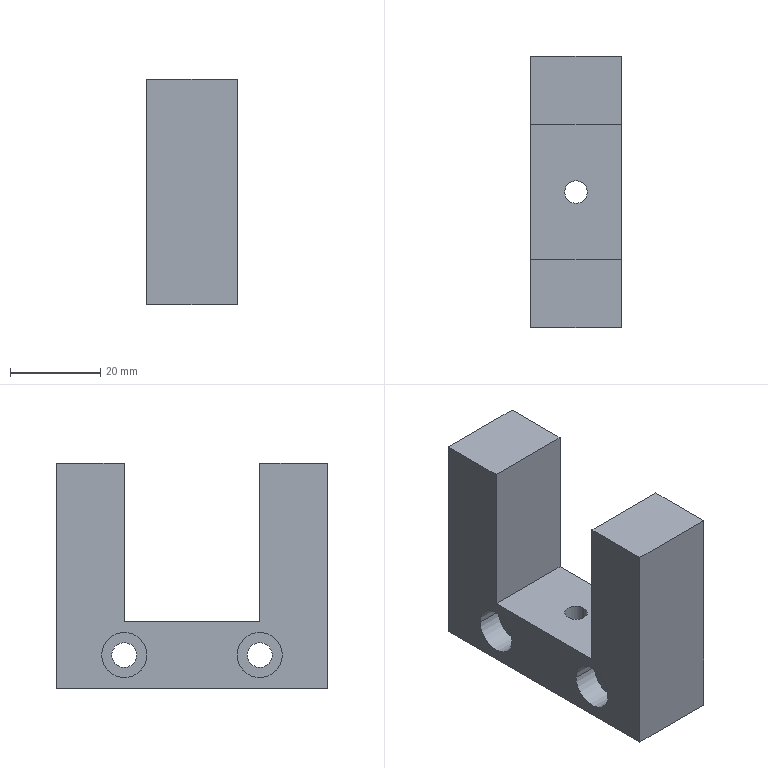Component | SolidWorks | LongSideClampingAssemblyBGeneralAssembly-1_LimitB-0510-1 | 1 solid | 22 faces | box 20 x 60 x 50 mm | volume 37131 mm3 | plane 12 | cylinder 10 | commonest cylinder face diameters 10 x4 5.5 x4 5 x2 | material Q235-A
build123d program:
from build123d import *

# Parameters (mm, degrees)
BOSS_EXTRUDE1_DEPTH                                = 20
HOLE_SIZE_ACCORDING_TO_TYPE_OF_HEX_SOC_D           = 5.5
HOLE_SIZE_ACCORDING_TO_TYPE_OF_HEX_SOC_CBORE_D     = 10
HOLE_SIZE_ACCORDING_TO_TYPE_OF_HEX_SOC_CBORE_DEPTH = 5.7
M6_TAPPED_HOLE1_D                                  = 5


with BuildPart() as part:
    # Sketch1 → Boss-Extrude1 (new body)
    with BuildSketch(Plane.XY):
        Polygon((-30, -25), (-15, -25), (-15, 10), (15, 10), (15, -25), (30, -25), (30, 25), (-30, 25), align=None)
    extrude(amount=BOSS_EXTRUDE1_DEPTH)

    # Hole Size _According to_ Type of Hex Soc (through all)
    with Locations(Plane.XY.offset(20)):
        with Locations((-15, 17.5), (15, 17.5)):
            CounterBoreHole(HOLE_SIZE_ACCORDING_TO_TYPE_OF_HEX_SOC_D / 2, HOLE_SIZE_ACCORDING_TO_TYPE_OF_HEX_SOC_CBORE_D / 2, HOLE_SIZE_ACCORDING_TO_TYPE_OF_HEX_SOC_CBORE_DEPTH)

    # M6 Tapped Hole1 (through all)
    with Locations(Plane(origin=(0, 25, 0), x_dir=(1, 0, 0), z_dir=(0, 1, 0))):
        with Locations((0, -10)):
            Hole(M6_TAPPED_HOLE1_D / 2)


solid = part.part

# Placed as in the assembly
solid = solid.moved(Location((-3220.658, 0.3914, 3511), (-90, -90, 0)))
STEP:
#1=CARTESIAN_POINT('',(-127.093,0.01541,137.835));
#2=VERTEX_POINT('',#1);
#3=CARTESIAN_POINT('',(-127.29,0.01541,137.835));
#4=VERTEX_POINT('',#3);
#5=CARTESIAN_POINT('',(-127.191,0.01541,137.835));
#6=DIRECTION('',(-0.,-0.,-1.));
#7=DIRECTION('',(0.,-1.,0.));
#8=AXIS2_PLACEMENT_3D('',#5,#6,#7);
#9=CIRCLE('',#8,0.09843);
#10=EDGE_CURVE('',#2,#4,#9,.T.);
#11=ORIENTED_EDGE('',*,*,#10,.F.);
#12=CARTESIAN_POINT('',(-127.093,0.01541,137.244));
#13=VERTEX_POINT('',#12);
#14=CARTESIAN_POINT('',(-127.093,0.01541,137.244));
#15=DIRECTION('',(-0.,-0.,-1.));
#16=VECTOR('',#15,39.37);
#17=LINE('',#14,#16);
#18=EDGE_CURVE('',#2,#13,#17,.T.);
#19=ORIENTED_EDGE('',*,*,#18,.T.);
#20=CARTESIAN_POINT('',(-127.29,0.01541,137.244));
#21=VERTEX_POINT('',#20);
#22=CARTESIAN_POINT('',(-127.191,0.01541,137.244));
#23=DIRECTION('',(-0.,-0.,-1.));
#24=DIRECTION('',(-1.,0.,0.));
#25=AXIS2_PLACEMENT_3D('',#22,#23,#24);
#26=CIRCLE('',#25,0.09843);
#27=EDGE_CURVE('',#13,#21,#26,.T.);
#28=ORIENTED_EDGE('',*,*,#27,.T.);
#29=CARTESIAN_POINT('',(-127.29,0.01541,137.244));
#30=DIRECTION('',(-0.,-0.,-1.));
#31=VECTOR('',#30,39.37);
#32=LINE('',#29,#31);
#33=EDGE_CURVE('',#4,#21,#32,.T.);
#34=ORIENTED_EDGE('',*,*,#33,.F.);
#35=EDGE_LOOP('',(#11,#19,#28,#34));
#36=FACE_OUTER_BOUND('',#35,.T.);
#37=CARTESIAN_POINT('',(-127.191,0.01541,137.244));
#38=DIRECTION('',(-0.,-0.,-1.));
#39=DIRECTION('',(-1.,0.,0.));
#40=AXIS2_PLACEMENT_3D('',#37,#38,#39);
#41=CYLINDRICAL_SURFACE('',#40,0.09843);
#42=ADVANCED_FACE('',(#36),#41,.F.);
#43=CARTESIAN_POINT('',(-127.361,-0.772,137.539));
#44=VERTEX_POINT('',#43);
#45=CARTESIAN_POINT('',(-127.361,-0.3783,137.539));
#46=VERTEX_POINT('',#45);
#47=CARTESIAN_POINT('',(-127.361,-0.5751,137.539));
#48=DIRECTION('',(-1.,0.,0.));
#49=DIRECTION('',(0.,1.,0.));
#50=AXIS2_PLACEMENT_3D('',#47,#48,#49);
#51=CIRCLE('',#50,0.1969);
#52=EDGE_CURVE('',#44,#46,#51,.T.);
#53=ORIENTED_EDGE('',*,*,#52,.F.);
#54=CARTESIAN_POINT('',(-127.585,-0.772,137.539));
#55=VERTEX_POINT('',#54);
#56=CARTESIAN_POINT('',(-127.585,-0.772,137.539));
#57=DIRECTION('',(-1.,0.,0.));
#58=VECTOR('',#57,39.37);
#59=LINE('',#56,#58);
#60=EDGE_CURVE('',#44,#55,#59,.T.);
#61=ORIENTED_EDGE('',*,*,#60,.T.);
#62=CARTESIAN_POINT('',(-127.585,-0.3783,137.539));
#63=VERTEX_POINT('',#62);
#64=CARTESIAN_POINT('',(-127.585,-0.5751,137.539));
#65=DIRECTION('',(-1.,0.,0.));
#66=DIRECTION('',(0.,1.,0.));
#67=AXIS2_PLACEMENT_3D('',#64,#65,#66);
#68=CIRCLE('',#67,0.1969);
#69=EDGE_CURVE('',#55,#63,#68,.T.);
#70=ORIENTED_EDGE('',*,*,#69,.T.);
#71=CARTESIAN_POINT('',(-127.585,-0.3783,137.539));
#72=DIRECTION('',(-1.,0.,0.));
#73=VECTOR('',#72,39.37);
#74=LINE('',#71,#73);
#75=EDGE_CURVE('',#46,#63,#74,.T.);
#76=ORIENTED_EDGE('',*,*,#75,.F.);
#77=EDGE_LOOP('',(#53,#61,#70,#76));
#78=FACE_OUTER_BOUND('',#77,.T.);
#79=CARTESIAN_POINT('',(-127.585,-0.5751,137.539));
#80=DIRECTION('',(-1.,0.,0.));
#81=DIRECTION('',(0.,1.,0.));
#82=AXIS2_PLACEMENT_3D('',#79,#80,#81);
#83=CYLINDRICAL_SURFACE('',#82,0.1969);
#84=ADVANCED_FACE('',(#78),#83,.F.);
#85=CARTESIAN_POINT('',(-126.798,-0.6834,137.539));
#86=VERTEX_POINT('',#85);
#87=CARTESIAN_POINT('',(-126.798,-0.4669,137.539));
#88=VERTEX_POINT('',#87);
#89=CARTESIAN_POINT('',(-126.798,-0.5751,137.539));
#90=DIRECTION('',(-1.,0.,0.));
#91=DIRECTION('',(0.,1.,0.));
#92=AXIS2_PLACEMENT_3D('',#89,#90,#91);
#93=CIRCLE('',#92,0.1083);
#94=EDGE_CURVE('',#86,#88,#93,.T.);
#95=ORIENTED_EDGE('',*,*,#94,.F.);
#96=CARTESIAN_POINT('',(-127.361,-0.6834,137.539));
#97=VERTEX_POINT('',#96);
#98=CARTESIAN_POINT('',(-127.585,-0.6834,137.539));
#99=DIRECTION('',(-1.,0.,0.));
#100=VECTOR('',#99,39.37);
#101=LINE('',#98,#100);
#102=EDGE_CURVE('',#86,#97,#101,.T.);
#103=ORIENTED_EDGE('',*,*,#102,.T.);
#104=CARTESIAN_POINT('',(-127.361,-0.4669,137.539));
#105=VERTEX_POINT('',#104);
#106=CARTESIAN_POINT('',(-127.361,-0.5751,137.539));
#107=DIRECTION('',(-1.,0.,0.));
#108=DIRECTION('',(0.,1.,0.));
#109=AXIS2_PLACEMENT_3D('',#106,#107,#108);
#110=CIRCLE('',#109,0.1083);
#111=EDGE_CURVE('',#97,#105,#110,.T.);
#112=ORIENTED_EDGE('',*,*,#111,.T.);
#113=CARTESIAN_POINT('',(-127.585,-0.4669,137.539));
#114=DIRECTION('',(-1.,0.,0.));
#115=VECTOR('',#114,39.37);
#116=LINE('',#113,#115);
#117=EDGE_CURVE('',#88,#105,#116,.T.);
#118=ORIENTED_EDGE('',*,*,#117,.F.);
#119=EDGE_LOOP('',(#95,#103,#112,#118));
#120=FACE_OUTER_BOUND('',#119,.T.);
#121=CARTESIAN_POINT('',(-127.585,-0.5751,137.539));
#122=DIRECTION('',(-1.,0.,0.));
#123=DIRECTION('',(0.,1.,0.));
#124=AXIS2_PLACEMENT_3D('',#121,#122,#123);
#125=CYLINDRICAL_SURFACE('',#124,0.1083);
#126=ADVANCED_FACE('',(#120),#125,.F.);
#127=CARTESIAN_POINT('',(-127.361,0.4091,137.539));
#128=VERTEX_POINT('',#127);
#129=CARTESIAN_POINT('',(-127.361,0.8028,137.539));
#130=VERTEX_POINT('',#129);
#131=CARTESIAN_POINT('',(-127.361,0.606,137.539));
#132=DIRECTION('',(-1.,0.,0.));
#133=DIRECTION('',(0.,1.,0.));
#134=AXIS2_PLACEMENT_3D('',#131,#132,#133);
#135=CIRCLE('',#134,0.1969);
#136=EDGE_CURVE('',#128,#130,#135,.T.);
#137=ORIENTED_EDGE('',*,*,#136,.F.);
#138=CARTESIAN_POINT('',(-127.585,0.4091,137.539));
#139=VERTEX_POINT('',#138);
#140=CARTESIAN_POINT('',(-127.585,0.4091,137.539));
#141=DIRECTION('',(-1.,0.,0.));
#142=VECTOR('',#141,39.37);
#143=LINE('',#140,#142);
#144=EDGE_CURVE('',#128,#139,#143,.T.);
#145=ORIENTED_EDGE('',*,*,#144,.T.);
#146=CARTESIAN_POINT('',(-127.585,0.8028,137.539));
#147=VERTEX_POINT('',#146);
#148=CARTESIAN_POINT('',(-127.585,0.606,137.539));
#149=DIRECTION('',(-1.,0.,0.));
#150=DIRECTION('',(0.,1.,0.));
#151=AXIS2_PLACEMENT_3D('',#148,#149,#150);
#152=CIRCLE('',#151,0.1969);
#153=EDGE_CURVE('',#139,#147,#152,.T.);
#154=ORIENTED_EDGE('',*,*,#153,.T.);
#155=CARTESIAN_POINT('',(-127.585,0.8028,137.539));
#156=DIRECTION('',(-1.,0.,0.));
#157=VECTOR('',#156,39.37);
#158=LINE('',#155,#157);
#159=EDGE_CURVE('',#130,#147,#158,.T.);
#160=ORIENTED_EDGE('',*,*,#159,.F.);
#161=EDGE_LOOP('',(#137,#145,#154,#160));
#162=FACE_OUTER_BOUND('',#161,.T.);
#163=CARTESIAN_POINT('',(-127.585,0.606,137.539));
#164=DIRECTION('',(-1.,0.,0.));
#165=DIRECTION('',(0.,1.,0.));
#166=AXIS2_PLACEMENT_3D('',#163,#164,#165);
#167=CYLINDRICAL_SURFACE('',#166,0.1969);
#168=ADVANCED_FACE('',(#162),#167,.F.);
#169=CARTESIAN_POINT('',(-126.798,0.4977,137.539));
#170=VERTEX_POINT('',#169);
#171=CARTESIAN_POINT('',(-126.798,0.7142,137.539));
#172=VERTEX_POINT('',#171);
#173=CARTESIAN_POINT('',(-126.798,0.606,137.539));
#174=DIRECTION('',(-1.,0.,0.));
#175=DIRECTION('',(0.,1.,0.));
#176=AXIS2_PLACEMENT_3D('',#173,#174,#175);
#177=CIRCLE('',#176,0.1083);
#178=EDGE_CURVE('',#170,#172,#177,.T.);
#179=ORIENTED_EDGE('',*,*,#178,.F.);
#180=CARTESIAN_POINT('',(-127.361,0.4977,137.539));
#181=VERTEX_POINT('',#180);
#182=CARTESIAN_POINT('',(-127.585,0.4977,137.539));
#183=DIRECTION('',(-1.,0.,0.));
#184=VECTOR('',#183,39.37);
#185=LINE('',#182,#184);
#186=EDGE_CURVE('',#170,#181,#185,.T.);
#187=ORIENTED_EDGE('',*,*,#186,.T.);
#188=CARTESIAN_POINT('',(-127.361,0.7142,137.539));
#189=VERTEX_POINT('',#188);
#190=CARTESIAN_POINT('',(-127.361,0.606,137.539));
#191=DIRECTION('',(-1.,0.,0.));
#192=DIRECTION('',(0.,1.,0.));
#193=AXIS2_PLACEMENT_3D('',#190,#191,#192);
#194=CIRCLE('',#193,0.1083);
#195=EDGE_CURVE('',#181,#189,#194,.T.);
#196=ORIENTED_EDGE('',*,*,#195,.T.);
#197=CARTESIAN_POINT('',(-127.585,0.7142,137.539));
#198=DIRECTION('',(-1.,0.,0.));
#199=VECTOR('',#198,39.37);
#200=LINE('',#197,#199);
#201=EDGE_CURVE('',#172,#189,#200,.T.);
#202=ORIENTED_EDGE('',*,*,#201,.F.);
#203=EDGE_LOOP('',(#179,#187,#196,#202));
#204=FACE_OUTER_BOUND('',#203,.T.);
#205=CARTESIAN_POINT('',(-127.585,0.606,137.539));
#206=DIRECTION('',(-1.,0.,0.));
#207=DIRECTION('',(0.,1.,0.));
#208=AXIS2_PLACEMENT_3D('',#205,#206,#207);
#209=CYLINDRICAL_SURFACE('',#208,0.1083);
#210=ADVANCED_FACE('',(#204),#209,.F.);
#211=CARTESIAN_POINT('',(-126.798,1.197,139.213));
#212=VERTEX_POINT('',#211);
#213=CARTESIAN_POINT('',(-126.798,1.197,137.244));
#214=VERTEX_POINT('',#213);
#215=CARTESIAN_POINT('',(-126.798,1.197,139.213));
#216=DIRECTION('',(-0.,0.,-1.));
#217=VECTOR('',#216,39.37);
#218=LINE('',#215,#217);
#219=EDGE_CURVE('',#212,#214,#218,.T.);
#220=ORIENTED_EDGE('',*,*,#219,.T.);
#221=CARTESIAN_POINT('',(-127.585,1.197,137.244));
#222=VERTEX_POINT('',#221);
#223=CARTESIAN_POINT('',(-127.585,1.197,137.244));
#224=DIRECTION('',(1.,-0.,-0.));
#225=VECTOR('',#224,39.37);
#226=LINE('',#223,#225);
#227=EDGE_CURVE('',#222,#214,#226,.T.);
#228=ORIENTED_EDGE('',*,*,#227,.F.);
#229=CARTESIAN_POINT('',(-127.585,1.197,139.213));
#230=VERTEX_POINT('',#229);
#231=CARTESIAN_POINT('',(-127.585,1.197,139.213));
#232=DIRECTION('',(-0.,0.,-1.));
#233=VECTOR('',#232,39.37);
#234=LINE('',#231,#233);
#235=EDGE_CURVE('',#230,#222,#234,.T.);
#236=ORIENTED_EDGE('',*,*,#235,.F.);
#237=CARTESIAN_POINT('',(-127.585,1.197,139.213));
#238=DIRECTION('',(1.,-0.,-0.));
#239=VECTOR('',#238,39.37);
#240=LINE('',#237,#239);
#241=EDGE_CURVE('',#230,#212,#240,.T.);
#242=ORIENTED_EDGE('',*,*,#241,.T.);
#243=EDGE_LOOP('',(#220,#228,#236,#242));
#244=FACE_OUTER_BOUND('',#243,.T.);
#245=CARTESIAN_POINT('',(-127.585,1.197,139.213));
#246=DIRECTION('',(-0.,-1.,-0.));
#247=DIRECTION('',(0.,-0.,1.));
#248=AXIS2_PLACEMENT_3D('',#245,#246,#247);
#249=PLANE('',#248);
#250=ADVANCED_FACE('',(#244),#249,.F.);
#251=CARTESIAN_POINT('',(-127.191,0.01541,137.244));
#252=DIRECTION('',(-0.,-0.,-1.));
#253=DIRECTION('',(-1.,0.,0.));
#254=AXIS2_PLACEMENT_3D('',#251,#252,#253);
#255=CIRCLE('',#254,0.09843);
#256=EDGE_CURVE('',#21,#13,#255,.T.);
#257=ORIENTED_EDGE('',*,*,#256,.F.);
#258=ORIENTED_EDGE('',*,*,#27,.F.);
#259=EDGE_LOOP('',(#257,#258));
#260=FACE_BOUND('',#259,.T.);
#261=CARTESIAN_POINT('',(-126.798,-1.166,137.244));
#262=VERTEX_POINT('',#261);
#263=CARTESIAN_POINT('',(-126.798,-1.166,137.244));
#264=DIRECTION('',(-0.,-1.,-0.));
#265=VECTOR('',#264,39.37);
#266=LINE('',#263,#265);
#267=EDGE_CURVE('',#214,#262,#266,.T.);
#268=ORIENTED_EDGE('',*,*,#267,.T.);
#269=CARTESIAN_POINT('',(-127.585,-1.166,137.244));
#270=VERTEX_POINT('',#269);
#271=CARTESIAN_POINT('',(-127.585,-1.166,137.244));
#272=DIRECTION('',(1.,-0.,-0.));
#273=VECTOR('',#272,39.37);
#274=LINE('',#271,#273);
#275=EDGE_CURVE('',#270,#262,#274,.T.);
#276=ORIENTED_EDGE('',*,*,#275,.F.);
#277=CARTESIAN_POINT('',(-127.585,-1.166,137.244));
#278=DIRECTION('',(-0.,-1.,-0.));
#279=VECTOR('',#278,39.37);
#280=LINE('',#277,#279);
#281=EDGE_CURVE('',#222,#270,#280,.T.);
#282=ORIENTED_EDGE('',*,*,#281,.F.);
#283=ORIENTED_EDGE('',*,*,#227,.T.);
#284=EDGE_LOOP('',(#268,#276,#282,#283));
#285=FACE_OUTER_BOUND('',#284,.T.);
#286=CARTESIAN_POINT('',(-127.585,-1.166,137.244));
#287=DIRECTION('',(0.,-0.,1.));
#288=DIRECTION('',(0.,1.,0.));
#289=AXIS2_PLACEMENT_3D('',#286,#287,#288);
#290=PLANE('',#289);
#291=ADVANCED_FACE('',(#260,#285),#290,.F.);
#292=CARTESIAN_POINT('',(-126.798,-1.166,139.213));
#293=VERTEX_POINT('',#292);
#294=CARTESIAN_POINT('',(-126.798,-1.166,139.213));
#295=DIRECTION('',(0.,-0.,1.));
#296=VECTOR('',#295,39.37);
#297=LINE('',#294,#296);
#298=EDGE_CURVE('',#262,#293,#297,.T.);
#299=ORIENTED_EDGE('',*,*,#298,.T.);
#300=CARTESIAN_POINT('',(-127.585,-1.166,139.213));
#301=VERTEX_POINT('',#300);
#302=CARTESIAN_POINT('',(-127.585,-1.166,139.213));
#303=DIRECTION('',(1.,-0.,-0.));
#304=VECTOR('',#303,39.37);
#305=LINE('',#302,#304);
#306=EDGE_CURVE('',#301,#293,#305,.T.);
#307=ORIENTED_EDGE('',*,*,#306,.F.);
#308=CARTESIAN_POINT('',(-127.585,-1.166,139.213));
#309=DIRECTION('',(0.,-0.,1.));
#310=VECTOR('',#309,39.37);
#311=LINE('',#308,#310);
#312=EDGE_CURVE('',#270,#301,#311,.T.);
#313=ORIENTED_EDGE('',*,*,#312,.F.);
#314=ORIENTED_EDGE('',*,*,#275,.T.);
#315=EDGE_LOOP('',(#299,#307,#313,#314));
#316=FACE_OUTER_BOUND('',#315,.T.);
#317=CARTESIAN_POINT('',(-127.585,-1.166,139.213));
#318=DIRECTION('',(0.,1.,0.));
#319=DIRECTION('',(-0.,0.,-1.));
#320=AXIS2_PLACEMENT_3D('',#317,#318,#319);
#321=PLANE('',#320);
#322=ADVANCED_FACE('',(#316),#321,.F.);
#323=CARTESIAN_POINT('',(-126.798,-0.5751,139.213));
#324=VERTEX_POINT('',#323);
#325=CARTESIAN_POINT('',(-126.798,-1.166,139.213));
#326=DIRECTION('',(0.,1.,-0.));
#327=VECTOR('',#326,39.37);
#328=LINE('',#325,#327);
#329=EDGE_CURVE('',#293,#324,#328,.T.);
#330=ORIENTED_EDGE('',*,*,#329,.T.);
#331=CARTESIAN_POINT('',(-127.585,-0.5751,139.213));
#332=VERTEX_POINT('',#331);
#333=CARTESIAN_POINT('',(-127.585,-0.5751,139.213));
#334=DIRECTION('',(1.,-0.,-0.));
#335=VECTOR('',#334,39.37);
#336=LINE('',#333,#335);
#337=EDGE_CURVE('',#332,#324,#336,.T.);
#338=ORIENTED_EDGE('',*,*,#337,.F.);
#339=CARTESIAN_POINT('',(-127.585,-1.166,139.213));
#340=DIRECTION('',(0.,1.,-0.));
#341=VECTOR('',#340,39.37);
#342=LINE('',#339,#341);
#343=EDGE_CURVE('',#301,#332,#342,.T.);
#344=ORIENTED_EDGE('',*,*,#343,.F.);
#345=ORIENTED_EDGE('',*,*,#306,.T.);
#346=EDGE_LOOP('',(#330,#338,#344,#345));
#347=FACE_OUTER_BOUND('',#346,.T.);
#348=CARTESIAN_POINT('',(-127.585,-1.166,139.213));
#349=DIRECTION('',(-0.,-0.,-1.));
#350=DIRECTION('',(-1.,0.,0.));
#351=AXIS2_PLACEMENT_3D('',#348,#349,#350);
#352=PLANE('',#351);
#353=ADVANCED_FACE('',(#347),#352,.F.);
#354=CARTESIAN_POINT('',(-126.798,-0.5751,137.835));
#355=VERTEX_POINT('',#354);
#356=CARTESIAN_POINT('',(-126.798,-0.5751,139.213));
#357=DIRECTION('',(-0.,-0.,-1.));
#358=VECTOR('',#357,39.37);
#359=LINE('',#356,#358);
#360=EDGE_CURVE('',#324,#355,#359,.T.);
#361=ORIENTED_EDGE('',*,*,#360,.T.);
#362=CARTESIAN_POINT('',(-127.585,-0.5751,137.835));
#363=VERTEX_POINT('',#362);
#364=CARTESIAN_POINT('',(-127.585,-0.5751,137.835));
#365=DIRECTION('',(1.,-0.,-0.));
#366=VECTOR('',#365,39.37);
#367=LINE('',#364,#366);
#368=EDGE_CURVE('',#363,#355,#367,.T.);
#369=ORIENTED_EDGE('',*,*,#368,.F.);
#370=CARTESIAN_POINT('',(-127.585,-0.5751,139.213));
#371=DIRECTION('',(-0.,-0.,-1.));
#372=VECTOR('',#371,39.37);
#373=LINE('',#370,#372);
#374=EDGE_CURVE('',#332,#363,#373,.T.);
#375=ORIENTED_EDGE('',*,*,#374,.F.);
#376=ORIENTED_EDGE('',*,*,#337,.T.);
#377=EDGE_LOOP('',(#361,#369,#375,#376));
#378=FACE_OUTER_BOUND('',#377,.T.);
#379=CARTESIAN_POINT('',(-127.585,-0.5751,139.213));
#380=DIRECTION('',(-0.,-1.,0.));
#381=DIRECTION('',(-1.,0.,0.));
#382=AXIS2_PLACEMENT_3D('',#379,#380,#381);
#383=PLANE('',#382);
#384=ADVANCED_FACE('',(#378),#383,.F.);
#385=CARTESIAN_POINT('',(-127.191,0.01541,137.835));
#386=DIRECTION('',(-0.,-0.,-1.));
#387=DIRECTION('',(0.,-1.,0.));
#388=AXIS2_PLACEMENT_3D('',#385,#386,#387);
#389=CIRCLE('',#388,0.09843);
#390=EDGE_CURVE('',#4,#2,#389,.T.);
#391=ORIENTED_EDGE('',*,*,#390,.T.);
#392=ORIENTED_EDGE('',*,*,#10,.T.);
#393=EDGE_LOOP('',(#391,#392));
#394=FACE_BOUND('',#393,.T.);
#395=CARTESIAN_POINT('',(-126.798,0.606,137.835));
#396=VERTEX_POINT('',#395);
#397=CARTESIAN_POINT('',(-126.798,-0.5751,137.835));
#398=DIRECTION('',(0.,1.,-0.));
#399=VECTOR('',#398,39.37);
#400=LINE('',#397,#399);
#401=EDGE_CURVE('',#355,#396,#400,.T.);
#402=ORIENTED_EDGE('',*,*,#401,.T.);
#403=CARTESIAN_POINT('',(-127.585,0.606,137.835));
#404=VERTEX_POINT('',#403);
#405=CARTESIAN_POINT('',(-127.585,0.606,137.835));
#406=DIRECTION('',(1.,-0.,-0.));
#407=VECTOR('',#406,39.37);
#408=LINE('',#405,#407);
#409=EDGE_CURVE('',#404,#396,#408,.T.);
#410=ORIENTED_EDGE('',*,*,#409,.F.);
#411=CARTESIAN_POINT('',(-127.585,-0.5751,137.835));
#412=DIRECTION('',(0.,1.,-0.));
#413=VECTOR('',#412,39.37);
#414=LINE('',#411,#413);
#415=EDGE_CURVE('',#363,#404,#414,.T.);
#416=ORIENTED_EDGE('',*,*,#415,.F.);
#417=ORIENTED_EDGE('',*,*,#368,.T.);
#418=EDGE_LOOP('',(#402,#410,#416,#417));
#419=FACE_OUTER_BOUND('',#418,.T.);
#420=CARTESIAN_POINT('',(-127.585,-0.5751,137.835));
#421=DIRECTION('',(-0.,-0.,-1.));
#422=DIRECTION('',(-0.,-1.,0.));
#423=AXIS2_PLACEMENT_3D('',#420,#421,#422);
#424=PLANE('',#423);
#425=ADVANCED_FACE('',(#394,#419),#424,.F.);
#426=CARTESIAN_POINT('',(-126.798,0.606,139.213));
#427=VERTEX_POINT('',#426);
#428=CARTESIAN_POINT('',(-126.798,0.606,139.213));
#429=DIRECTION('',(0.,0.,1.));
#430=VECTOR('',#429,39.37);
#431=LINE('',#428,#430);
#432=EDGE_CURVE('',#396,#427,#431,.T.);
#433=ORIENTED_EDGE('',*,*,#432,.T.);
#434=CARTESIAN_POINT('',(-127.585,0.606,139.213));
#435=VERTEX_POINT('',#434);
#436=CARTESIAN_POINT('',(-127.585,0.606,139.213));
#437=DIRECTION('',(1.,-0.,-0.));
#438=VECTOR('',#437,39.37);
#439=LINE('',#436,#438);
#440=EDGE_CURVE('',#435,#427,#439,.T.);
#441=ORIENTED_EDGE('',*,*,#440,.F.);
#442=CARTESIAN_POINT('',(-127.585,0.606,139.213));
#443=DIRECTION('',(0.,0.,1.));
#444=VECTOR('',#443,39.37);
#445=LINE('',#442,#444);
#446=EDGE_CURVE('',#404,#435,#445,.T.);
#447=ORIENTED_EDGE('',*,*,#446,.F.);
#448=ORIENTED_EDGE('',*,*,#409,.T.);
#449=EDGE_LOOP('',(#433,#441,#447,#448));
#450=FACE_OUTER_BOUND('',#449,.T.);
#451=CARTESIAN_POINT('',(-127.585,0.606,139.213));
#452=DIRECTION('',(0.,1.,-0.));
#453=DIRECTION('',(-0.,-0.,-1.));
#454=AXIS2_PLACEMENT_3D('',#451,#452,#453);
#455=PLANE('',#454);
#456=ADVANCED_FACE('',(#450),#455,.F.);
#457=CARTESIAN_POINT('',(-126.798,0.606,139.213));
#458=DIRECTION('',(0.,1.,0.));
#459=VECTOR('',#458,39.37);
#460=LINE('',#457,#459);
#461=EDGE_CURVE('',#427,#212,#460,.T.);
#462=ORIENTED_EDGE('',*,*,#461,.T.);
#463=ORIENTED_EDGE('',*,*,#241,.F.);
#464=CARTESIAN_POINT('',(-127.585,0.606,139.213));
#465=DIRECTION('',(0.,1.,0.));
#466=VECTOR('',#465,39.37);
#467=LINE('',#464,#466);
#468=EDGE_CURVE('',#435,#230,#467,.T.);
#469=ORIENTED_EDGE('',*,*,#468,.F.);
#470=ORIENTED_EDGE('',*,*,#440,.T.);
#471=EDGE_LOOP('',(#462,#463,#469,#470));
#472=FACE_OUTER_BOUND('',#471,.T.);
#473=CARTESIAN_POINT('',(-127.585,0.606,139.213));
#474=DIRECTION('',(-0.,0.,-1.));
#475=DIRECTION('',(-0.,-1.,-0.));
#476=AXIS2_PLACEMENT_3D('',#473,#474,#475);
#477=PLANE('',#476);
#478=ADVANCED_FACE('',(#472),#477,.F.);
#479=CARTESIAN_POINT('',(-127.585,-0.5751,137.539));
#480=DIRECTION('',(-1.,0.,0.));
#481=DIRECTION('',(0.,1.,0.));
#482=AXIS2_PLACEMENT_3D('',#479,#480,#481);
#483=CIRCLE('',#482,0.1969);
#484=EDGE_CURVE('',#63,#55,#483,.T.);
#485=ORIENTED_EDGE('',*,*,#484,.F.);
#486=ORIENTED_EDGE('',*,*,#69,.F.);
#487=EDGE_LOOP('',(#485,#486));
#488=FACE_BOUND('',#487,.T.);
#489=CARTESIAN_POINT('',(-127.585,0.606,137.539));
#490=DIRECTION('',(-1.,0.,0.));
#491=DIRECTION('',(0.,1.,0.));
#492=AXIS2_PLACEMENT_3D('',#489,#490,#491);
#493=CIRCLE('',#492,0.1969);
#494=EDGE_CURVE('',#147,#139,#493,.T.);
#495=ORIENTED_EDGE('',*,*,#494,.F.);
#496=ORIENTED_EDGE('',*,*,#153,.F.);
#497=EDGE_LOOP('',(#495,#496));
#498=FACE_BOUND('',#497,.T.);
#499=ORIENTED_EDGE('',*,*,#235,.T.);
#500=ORIENTED_EDGE('',*,*,#281,.T.);
#501=ORIENTED_EDGE('',*,*,#312,.T.);
#502=ORIENTED_EDGE('',*,*,#343,.T.);
#503=ORIENTED_EDGE('',*,*,#374,.T.);
#504=ORIENTED_EDGE('',*,*,#415,.T.);
#505=ORIENTED_EDGE('',*,*,#446,.T.);
#506=ORIENTED_EDGE('',*,*,#468,.T.);
#507=EDGE_LOOP('',(#499,#500,#501,#502,#503,#504,#505,#506));
#508=FACE_OUTER_BOUND('',#507,.T.);
#509=CARTESIAN_POINT('',(-127.585,0.01541,138.228));
#510=DIRECTION('',(1.,-0.,-0.));
#511=DIRECTION('',(-0.,-1.,0.));
#512=AXIS2_PLACEMENT_3D('',#509,#510,#511);
#513=PLANE('',#512);
#514=ADVANCED_FACE('',(#488,#498,#508),#513,.F.);
#515=CARTESIAN_POINT('',(-126.798,-0.5751,137.539));
#516=DIRECTION('',(-1.,0.,0.));
#517=DIRECTION('',(0.,1.,0.));
#518=AXIS2_PLACEMENT_3D('',#515,#516,#517);
#519=CIRCLE('',#518,0.1083);
#520=EDGE_CURVE('',#88,#86,#519,.T.);
#521=ORIENTED_EDGE('',*,*,#520,.T.);
#522=ORIENTED_EDGE('',*,*,#94,.T.);
#523=EDGE_LOOP('',(#521,#522));
#524=FACE_BOUND('',#523,.T.);
#525=CARTESIAN_POINT('',(-126.798,0.606,137.539));
#526=DIRECTION('',(-1.,0.,0.));
#527=DIRECTION('',(0.,1.,0.));
#528=AXIS2_PLACEMENT_3D('',#525,#526,#527);
#529=CIRCLE('',#528,0.1083);
#530=EDGE_CURVE('',#172,#170,#529,.T.);
#531=ORIENTED_EDGE('',*,*,#530,.T.);
#532=ORIENTED_EDGE('',*,*,#178,.T.);
#533=EDGE_LOOP('',(#531,#532));
#534=FACE_BOUND('',#533,.T.);
#535=ORIENTED_EDGE('',*,*,#219,.F.);
#536=ORIENTED_EDGE('',*,*,#461,.F.);
#537=ORIENTED_EDGE('',*,*,#432,.F.);
#538=ORIENTED_EDGE('',*,*,#401,.F.);
#539=ORIENTED_EDGE('',*,*,#360,.F.);
#540=ORIENTED_EDGE('',*,*,#329,.F.);
#541=ORIENTED_EDGE('',*,*,#298,.F.);
#542=ORIENTED_EDGE('',*,*,#267,.F.);
#543=EDGE_LOOP('',(#535,#536,#537,#538,#539,#540,#541,#542));
#544=FACE_OUTER_BOUND('',#543,.T.);
#545=CARTESIAN_POINT('',(-126.798,0.01541,138.228));
#546=DIRECTION('',(1.,-0.,-0.));
#547=DIRECTION('',(-0.,-1.,0.));
#548=AXIS2_PLACEMENT_3D('',#545,#546,#547);
#549=PLANE('',#548);
#550=ADVANCED_FACE('',(#524,#534,#544),#549,.T.);
#551=ORIENTED_EDGE('',*,*,#186,.F.);
#552=ORIENTED_EDGE('',*,*,#530,.F.);
#553=ORIENTED_EDGE('',*,*,#201,.T.);
#554=CARTESIAN_POINT('',(-127.361,0.606,137.539));
#555=DIRECTION('',(-1.,0.,0.));
#556=DIRECTION('',(0.,1.,0.));
#557=AXIS2_PLACEMENT_3D('',#554,#555,#556);
#558=CIRCLE('',#557,0.1083);
#559=EDGE_CURVE('',#189,#181,#558,.T.);
#560=ORIENTED_EDGE('',*,*,#559,.T.);
#561=EDGE_LOOP('',(#551,#552,#553,#560));
#562=FACE_OUTER_BOUND('',#561,.T.);
#563=CARTESIAN_POINT('',(-127.585,0.606,137.539));
#564=DIRECTION('',(-1.,0.,0.));
#565=DIRECTION('',(0.,1.,0.));
#566=AXIS2_PLACEMENT_3D('',#563,#564,#565);
#567=CYLINDRICAL_SURFACE('',#566,0.1083);
#568=ADVANCED_FACE('',(#562),#567,.F.);
#569=ORIENTED_EDGE('',*,*,#559,.F.);
#570=ORIENTED_EDGE('',*,*,#195,.F.);
#571=EDGE_LOOP('',(#569,#570));
#572=FACE_BOUND('',#571,.T.);
#573=CARTESIAN_POINT('',(-127.361,0.606,137.539));
#574=DIRECTION('',(-1.,0.,0.));
#575=DIRECTION('',(0.,1.,0.));
#576=AXIS2_PLACEMENT_3D('',#573,#574,#575);
#577=CIRCLE('',#576,0.1969);
#578=EDGE_CURVE('',#130,#128,#577,.T.);
#579=ORIENTED_EDGE('',*,*,#578,.T.);
#580=ORIENTED_EDGE('',*,*,#136,.T.);
#581=EDGE_LOOP('',(#579,#580));
#582=FACE_OUTER_BOUND('',#581,.T.);
#583=CARTESIAN_POINT('',(-127.361,0.7142,137.539));
#584=DIRECTION('',(1.,-0.,-0.));
#585=DIRECTION('',(-0.,-1.,0.));
#586=AXIS2_PLACEMENT_3D('',#583,#584,#585);
#587=PLANE('',#586);
#588=ADVANCED_FACE('',(#572,#582),#587,.F.);
#589=ORIENTED_EDGE('',*,*,#144,.F.);
#590=ORIENTED_EDGE('',*,*,#578,.F.);
#591=ORIENTED_EDGE('',*,*,#159,.T.);
#592=ORIENTED_EDGE('',*,*,#494,.T.);
#593=EDGE_LOOP('',(#589,#590,#591,#592));
#594=FACE_OUTER_BOUND('',#593,.T.);
#595=CARTESIAN_POINT('',(-127.585,0.606,137.539));
#596=DIRECTION('',(-1.,0.,0.));
#597=DIRECTION('',(0.,1.,0.));
#598=AXIS2_PLACEMENT_3D('',#595,#596,#597);
#599=CYLINDRICAL_SURFACE('',#598,0.1969);
#600=ADVANCED_FACE('',(#594),#599,.F.);
#601=ORIENTED_EDGE('',*,*,#102,.F.);
#602=ORIENTED_EDGE('',*,*,#520,.F.);
#603=ORIENTED_EDGE('',*,*,#117,.T.);
#604=CARTESIAN_POINT('',(-127.361,-0.5751,137.539));
#605=DIRECTION('',(-1.,0.,0.));
#606=DIRECTION('',(0.,1.,0.));
#607=AXIS2_PLACEMENT_3D('',#604,#605,#606);
#608=CIRCLE('',#607,0.1083);
#609=EDGE_CURVE('',#105,#97,#608,.T.);
#610=ORIENTED_EDGE('',*,*,#609,.T.);
#611=EDGE_LOOP('',(#601,#602,#603,#610));
#612=FACE_OUTER_BOUND('',#611,.T.);
#613=CARTESIAN_POINT('',(-127.585,-0.5751,137.539));
#614=DIRECTION('',(-1.,0.,0.));
#615=DIRECTION('',(0.,1.,0.));
#616=AXIS2_PLACEMENT_3D('',#613,#614,#615);
#617=CYLINDRICAL_SURFACE('',#616,0.1083);
#618=ADVANCED_FACE('',(#612),#617,.F.);
#619=ORIENTED_EDGE('',*,*,#609,.F.);
#620=ORIENTED_EDGE('',*,*,#111,.F.);
#621=EDGE_LOOP('',(#619,#620));
#622=FACE_BOUND('',#621,.T.);
#623=CARTESIAN_POINT('',(-127.361,-0.5751,137.539));
#624=DIRECTION('',(-1.,0.,0.));
#625=DIRECTION('',(0.,1.,0.));
#626=AXIS2_PLACEMENT_3D('',#623,#624,#625);
#627=CIRCLE('',#626,0.1969);
#628=EDGE_CURVE('',#46,#44,#627,.T.);
#629=ORIENTED_EDGE('',*,*,#628,.T.);
#630=ORIENTED_EDGE('',*,*,#52,.T.);
#631=EDGE_LOOP('',(#629,#630));
#632=FACE_OUTER_BOUND('',#631,.T.);
#633=CARTESIAN_POINT('',(-127.361,-0.4669,137.539));
#634=DIRECTION('',(1.,-0.,-0.));
#635=DIRECTION('',(-0.,-1.,0.));
#636=AXIS2_PLACEMENT_3D('',#633,#634,#635);
#637=PLANE('',#636);
#638=ADVANCED_FACE('',(#622,#632),#637,.F.);
#639=ORIENTED_EDGE('',*,*,#60,.F.);
#640=ORIENTED_EDGE('',*,*,#628,.F.);
#641=ORIENTED_EDGE('',*,*,#75,.T.);
#642=ORIENTED_EDGE('',*,*,#484,.T.);
#643=EDGE_LOOP('',(#639,#640,#641,#642));
#644=FACE_OUTER_BOUND('',#643,.T.);
#645=CARTESIAN_POINT('',(-127.585,-0.5751,137.539));
#646=DIRECTION('',(-1.,0.,0.));
#647=DIRECTION('',(0.,1.,0.));
#648=AXIS2_PLACEMENT_3D('',#645,#646,#647);
#649=CYLINDRICAL_SURFACE('',#648,0.1969);
#650=ADVANCED_FACE('',(#644),#649,.F.);
#651=ORIENTED_EDGE('',*,*,#18,.F.);
#652=ORIENTED_EDGE('',*,*,#390,.F.);
#653=ORIENTED_EDGE('',*,*,#33,.T.);
#654=ORIENTED_EDGE('',*,*,#256,.T.);
#655=EDGE_LOOP('',(#651,#652,#653,#654));
#656=FACE_OUTER_BOUND('',#655,.T.);
#657=CARTESIAN_POINT('',(-127.191,0.01541,137.244));
#658=DIRECTION('',(-0.,-0.,-1.));
#659=DIRECTION('',(-1.,0.,0.));
#660=AXIS2_PLACEMENT_3D('',#657,#658,#659);
#661=CYLINDRICAL_SURFACE('',#660,0.09843);
#662=ADVANCED_FACE('',(#656),#661,.F.);
#663=CLOSED_SHELL('',(#42,#84,#126,#168,#210,#250,#291,#322,#353,#384,#425,#456,#478,#514,#550,#568,#588,#600,#618,#638,#650,#662));
#664=MANIFOLD_SOLID_BREP('',#663);
#665=CARTESIAN_POINT('',(0.,0.,0.));
#666=DIRECTION('',(0.,0.,1.));
#667=DIRECTION('',(1.,0.,0.));
#668=AXIS2_PLACEMENT_3D('',#665,#666,#667);
#669=(LENGTH_UNIT()NAMED_UNIT(*)SI_UNIT($,.METRE.));
#670=LENGTH_MEASURE_WITH_UNIT(LENGTH_MEASURE(0.0254),#669);
#671=DIMENSIONAL_EXPONENTS(1.,0.,0.,0.,0.,0.,0.);
#672=(CONVERSION_BASED_UNIT('',#670)LENGTH_UNIT()NAMED_UNIT(#671));
#673=UNCERTAINTY_MEASURE_WITH_UNIT(LENGTH_MEASURE(0.00001),#672,'','');
#674=(NAMED_UNIT(*)PLANE_ANGLE_UNIT()SI_UNIT($,.RADIAN.));
#675=(NAMED_UNIT(*)SI_UNIT($,.STERADIAN.)SOLID_ANGLE_UNIT());
#676=(GEOMETRIC_REPRESENTATION_CONTEXT(3)GLOBAL_UNCERTAINTY_ASSIGNED_CONTEXT((#673))GLOBAL_UNIT_ASSIGNED_CONTEXT((#672,#674,#675))REPRESENTATION_CONTEXT('',''));
#677=ADVANCED_BREP_SHAPE_REPRESENTATION('',(#664,#668),#676);
#678=COLOUR_RGB('',0.7922,0.8196,0.9333);
#679=FILL_AREA_STYLE_COLOUR('',#678);
#680=FILL_AREA_STYLE('',(#679));
#681=SURFACE_STYLE_FILL_AREA(#680);
#682=SURFACE_SIDE_STYLE('',(#681));
#683=SURFACE_STYLE_USAGE(.BOTH.,#682);
#684=PRESENTATION_STYLE_ASSIGNMENT((#683));
#685=STYLED_ITEM('',(#684),#664);
#686=PRESENTATION_LAYER_ASSIGNMENT('','',(#685));
#687=(LENGTH_UNIT()NAMED_UNIT(*)SI_UNIT($,.METRE.));
#688=LENGTH_MEASURE_WITH_UNIT(LENGTH_MEASURE(0.0254),#687);
#689=DIMENSIONAL_EXPONENTS(1.,0.,0.,0.,0.,0.,0.);
#690=(CONVERSION_BASED_UNIT('',#688)LENGTH_UNIT()NAMED_UNIT(#689));
#691=UNCERTAINTY_MEASURE_WITH_UNIT(LENGTH_MEASURE(0.00001),#690,'','');
#692=(NAMED_UNIT(*)PLANE_ANGLE_UNIT()SI_UNIT($,.RADIAN.));
#693=(NAMED_UNIT(*)SI_UNIT($,.STERADIAN.)SOLID_ANGLE_UNIT());
#694=(GEOMETRIC_REPRESENTATION_CONTEXT(3)GLOBAL_UNCERTAINTY_ASSIGNED_CONTEXT((#691))GLOBAL_UNIT_ASSIGNED_CONTEXT((#690,#692,#693))REPRESENTATION_CONTEXT('',''));
#695=MECHANICAL_DESIGN_GEOMETRIC_PRESENTATION_REPRESENTATION('',(#685),#694);